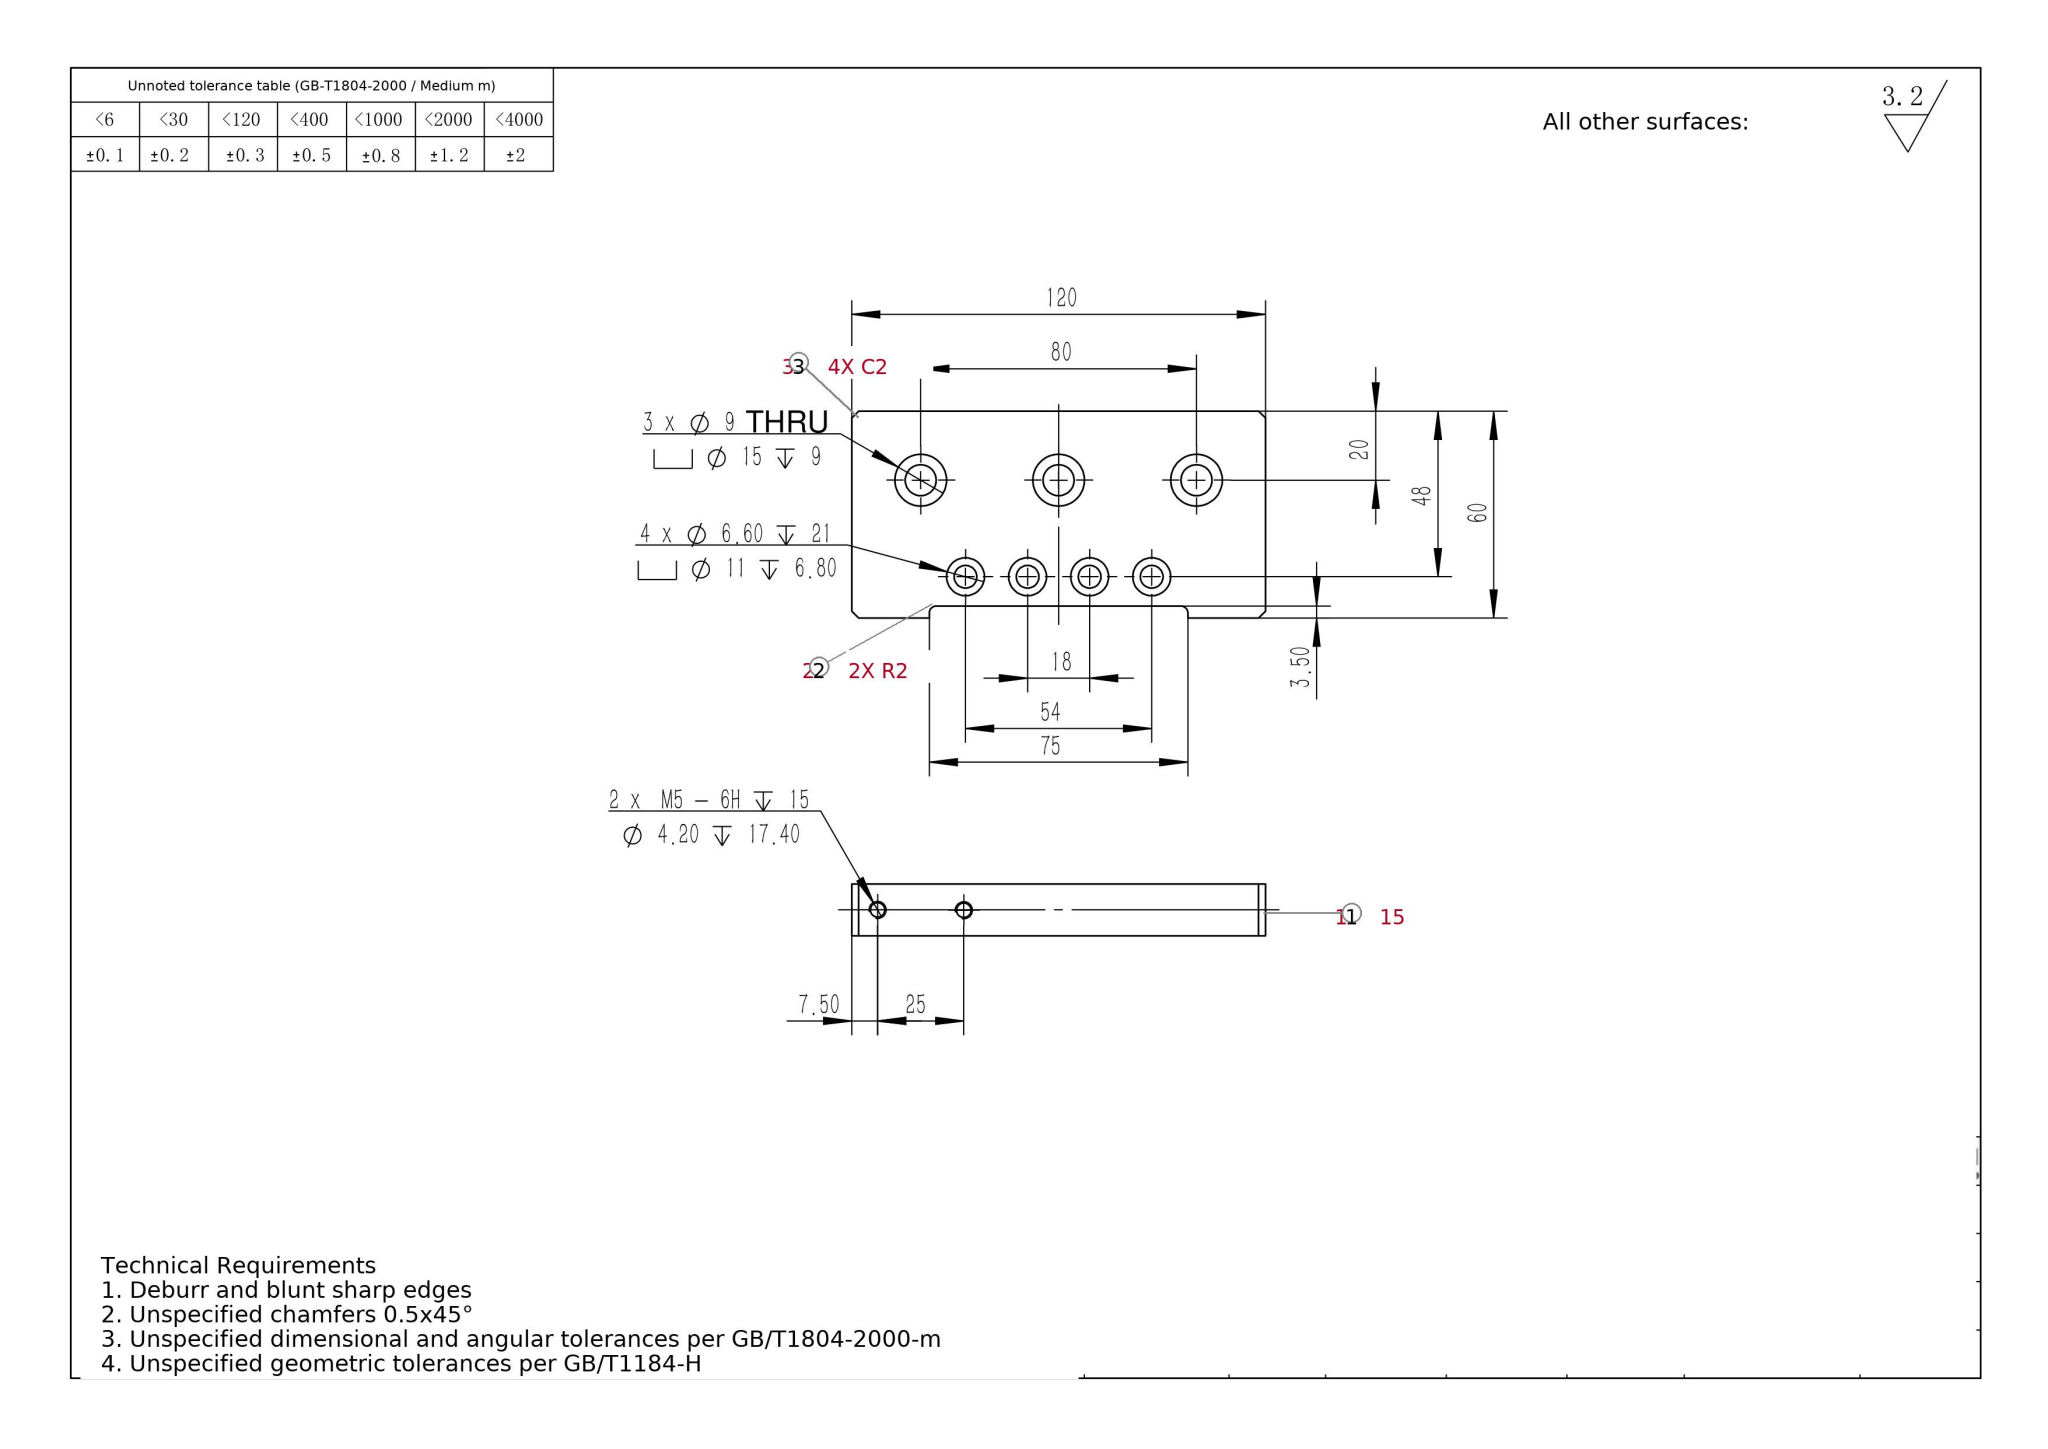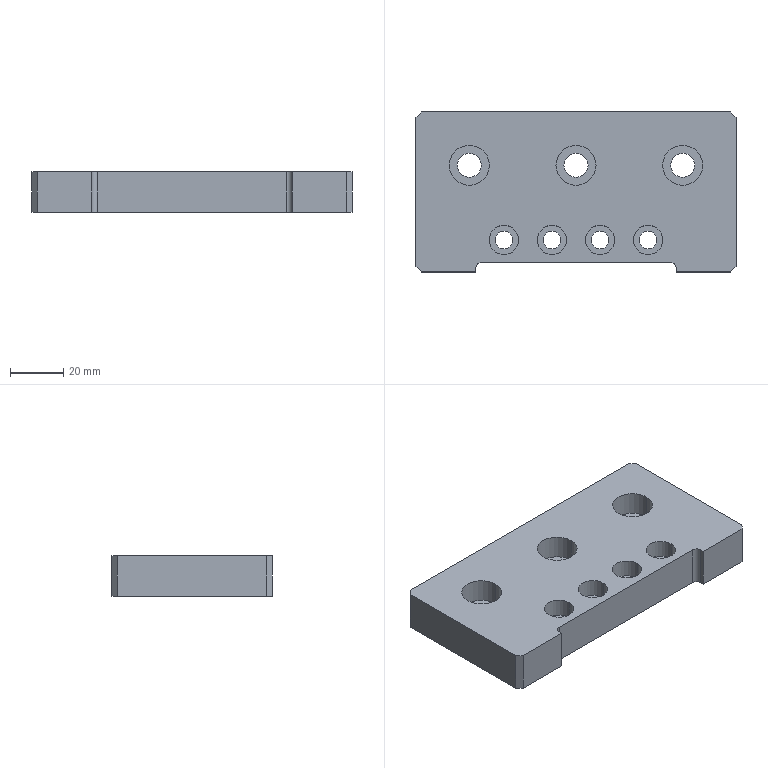Part | SolidWorks | mm | 1 solid | 59 faces | box 120 x 60 x 15 mm | volume 93851 mm3 | cylinder 34 | plane 21 | cone 4 | commonest cylinder face diameters 11 x8 6.6 x8 15 x6 9 x6 4.2 x4 4 x2
build123d program:
from build123d import *

# Parameters (mm, degrees)
SKETCH1_W                                         = 120
SKETCH1_H                                         = 60
BOSS_EXTRUDE1_DEPTH                               = 15
SKETCH2_W                                         = 75
SKETCH2_H                                         = 3.5
CUT_EXTRUDE1_DEPTH                                = 69.739
CHAMFER1_SIZE                                     = 2
HOLE_SIZE_ACCORDING_TO_HEX_SOCKET_HEA_D           = 6.6
HOLE_SIZE_ACCORDING_TO_HEX_SOCKET_HEA_DEPTH       = 21
HOLE_SIZE_ACCORDING_TO_HEX_SOCKET_HEA_CBORE_D     = 11
HOLE_SIZE_ACCORDING_TO_HEX_SOCKET_HEA_CBORE_DEPTH = 6.8
HOLE_SIZE_ACCORDING_TO_HEX_SOCKET_HEA_TIP         = 1.983
FILLET1_R                                         = 2
HOLE_SIZE_ACCORDING_TO_HEX_SOCKET_2_D             = 9
HOLE_SIZE_ACCORDING_TO_HEX_SOCKET_2_CBORE_D       = 15
HOLE_SIZE_ACCORDING_TO_HEX_SOCKET_2_CBORE_DEPTH   = 9
M5_TAPPED_HOLE1_D                                 = 4.2
M5_TAPPED_HOLE1_DEPTH                             = 17.4
M5_TAPPED_HOLE1_TIP                               = 1.262


with BuildPart() as part:
    # Sketch1 → Boss-Extrude1 (new body)
    with BuildSketch(Plane.XY):
        Rectangle(SKETCH1_W, SKETCH1_H)
    extrude(amount=BOSS_EXTRUDE1_DEPTH)

    # Sketch2 → Cut-Extrude1 (cut, through all)
    with BuildSketch(Plane.XY.offset(15)):
        with Locations((0, -28.25)):
            Rectangle(SKETCH2_W, SKETCH2_H)
    extrude(amount=-CUT_EXTRUDE1_DEPTH, mode=Mode.SUBTRACT)

    # Chamfer1
    chamfer1_edges = [part.edges().sort_by_distance(p)[0] for p in [
        (60, -30, 7.5),
        (-60, -30, 7.5),
        (-60, 30, 7.5),
        (60, 30, 7.5),
    ]]
    chamfer(chamfer1_edges, length=CHAMFER1_SIZE)

    # Hole Size _ according to_ Hex Socket Hea
    with Locations(Plane.XY.offset(15)):
        with Locations((27, -18), (9, -18), (-9, -18), (-27, -18)):
            CounterBoreHole(HOLE_SIZE_ACCORDING_TO_HEX_SOCKET_HEA_D / 2, HOLE_SIZE_ACCORDING_TO_HEX_SOCKET_HEA_CBORE_D / 2, HOLE_SIZE_ACCORDING_TO_HEX_SOCKET_HEA_CBORE_DEPTH, depth=HOLE_SIZE_ACCORDING_TO_HEX_SOCKET_HEA_DEPTH)
            with Locations((0, 0, -(HOLE_SIZE_ACCORDING_TO_HEX_SOCKET_HEA_DEPTH + HOLE_SIZE_ACCORDING_TO_HEX_SOCKET_HEA_TIP / 2))):  # 118° drill point
                Cone(0, HOLE_SIZE_ACCORDING_TO_HEX_SOCKET_HEA_D / 2, HOLE_SIZE_ACCORDING_TO_HEX_SOCKET_HEA_TIP, mode=Mode.SUBTRACT)

    # Fillet1
    fillet1_edges = [part.edges().sort_by_distance(p)[0] for p in [
        (37.5, -26.5, 7.5),
        (-37.5, -26.5, 7.5),
    ]]
    fillet(fillet1_edges, radius=FILLET1_R)

    # Hole Size _ according to_ Hex Socket 2 (through all)
    with Locations(Plane.XY.offset(15)):
        with Locations((40, 10), (0, 10), (-40, 10)):
            CounterBoreHole(HOLE_SIZE_ACCORDING_TO_HEX_SOCKET_2_D / 2, HOLE_SIZE_ACCORDING_TO_HEX_SOCKET_2_CBORE_D / 2, HOLE_SIZE_ACCORDING_TO_HEX_SOCKET_2_CBORE_DEPTH)

    # M5 Tapped Hole1
    with Locations(Plane(origin=(0, 30, 0), x_dir=(1, 0, 0), z_dir=(0, 1, 0))):
        with Locations((-27.5, -7.598), (-52.5, -7.5)):
            Hole(M5_TAPPED_HOLE1_D / 2, depth=M5_TAPPED_HOLE1_DEPTH)
            with Locations((0, 0, -(M5_TAPPED_HOLE1_DEPTH + M5_TAPPED_HOLE1_TIP / 2))):  # 118° drill point
                Cone(0, M5_TAPPED_HOLE1_D / 2, M5_TAPPED_HOLE1_TIP, mode=Mode.SUBTRACT)


solid = part.part